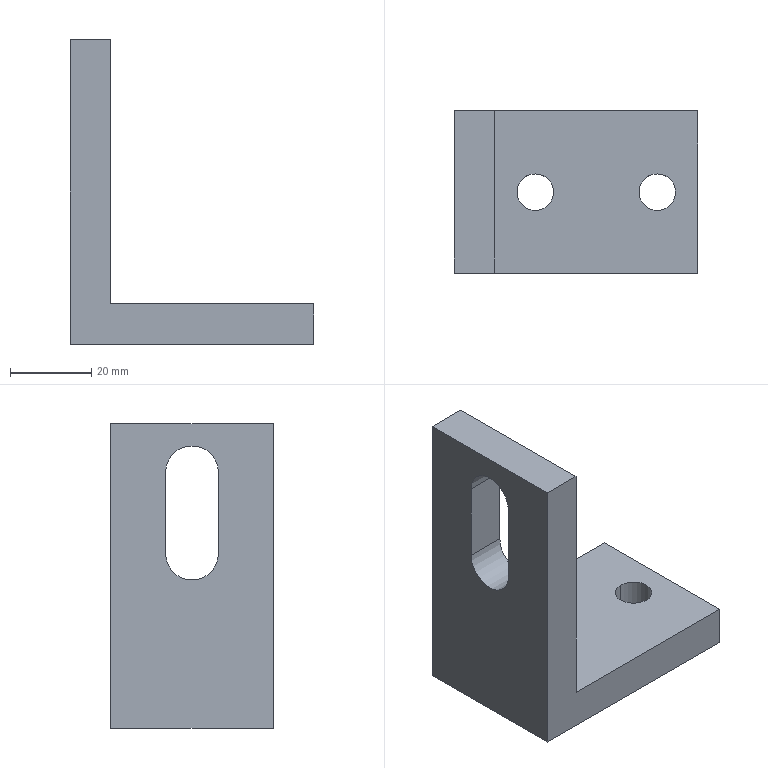Component | SolidWorks | KSD171005A-01-01-44-1 | 1 solid | 16 faces | box 60 x 40 x 75 mm | volume 44800 mm3 | plane 10 | cylinder 6 | commonest cylinder face diameters 9 x4 13 x2
build123d program:
from build123d import *

# Parameters (mm, degrees)
BOSS_EXTRUDE1_DEPTH      = 40
F_9_0_9_DIAMETER_HOLE1_D = 9
CUT_EXTRUDE1_DEPTH       = 105.043


with BuildPart() as part:
    # Sketch1 → Boss-Extrude1 (new body)
    with BuildSketch(Plane.XY):
        Polygon((0, 0), (75, 0), (75, -10), (10, -10), (10, -60), (0, -60), align=None)
    extrude(amount=BOSS_EXTRUDE1_DEPTH)

    # 9.0 _9_ Diameter Hole1 (through all)
    with Locations(Plane(origin=(10, 0, 0), x_dir=(0, 0, -1), z_dir=(1, 0, 0))):
        with Locations((-20, -20), (-20, -50)):
            Hole(F_9_0_9_DIAMETER_HOLE1_D / 2)

    # Sketch4 → Cut-Extrude1 (cut, through all)
    with BuildSketch(Plane(origin=(0, 0, 0), x_dir=(1, 0, 0), z_dir=(0, 1, 0))):
        with BuildLine():
            Line((63, -26.5), (43, -26.5))
            ThreePointArc((43, -26.5), (36.5, -20), (43, -13.5))
            Line((43, -13.5), (63, -13.5))
            ThreePointArc((63, -13.5), (69.5, -20), (63, -26.5))
        make_face()
    extrude(amount=-CUT_EXTRUDE1_DEPTH, mode=Mode.SUBTRACT)


solid = part.part

# Placed as in the assembly
solid = solid.moved(Location((32.889, -4.27, 568), (90, 0, 90)))
STEP:
#1=COLOUR_RGB('',0.7922,0.8196,0.9333);
#2=FILL_AREA_STYLE_COLOUR('',#1);
#3=FILL_AREA_STYLE('',(#2));
#4=SURFACE_STYLE_FILL_AREA(#3);
#5=SURFACE_SIDE_STYLE('',(#4));
#6=SURFACE_STYLE_USAGE(.BOTH.,#5);
#7=PRESENTATION_STYLE_ASSIGNMENT((#6));
#8=CARTESIAN_POINT('',(2.082,-1.133,22.362));
#9=VERTEX_POINT('',#8);
#10=CARTESIAN_POINT('',(2.082,-0.7784,22.362));
#11=VERTEX_POINT('',#10);
#12=CARTESIAN_POINT('',(2.082,-0.9555,22.362));
#13=DIRECTION('',(0.,0.,1.));
#14=DIRECTION('',(0.,1.,0.));
#15=AXIS2_PLACEMENT_3D('',#12,#13,#14);
#16=CIRCLE('',#15,0.1772);
#17=EDGE_CURVE('',#9,#11,#16,.T.);
#18=ORIENTED_EDGE('',*,*,#17,.F.);
#19=CARTESIAN_POINT('',(2.082,-1.133,22.756));
#20=VERTEX_POINT('',#19);
#21=CARTESIAN_POINT('',(2.082,-1.133,22.756));
#22=DIRECTION('',(0.,0.,1.));
#23=VECTOR('',#22,39.37);
#24=LINE('',#21,#23);
#25=EDGE_CURVE('',#9,#20,#24,.T.);
#26=ORIENTED_EDGE('',*,*,#25,.T.);
#27=CARTESIAN_POINT('',(2.082,-0.7784,22.756));
#28=VERTEX_POINT('',#27);
#29=CARTESIAN_POINT('',(2.082,-0.9555,22.756));
#30=DIRECTION('',(0.,0.,1.));
#31=DIRECTION('',(0.,1.,0.));
#32=AXIS2_PLACEMENT_3D('',#29,#30,#31);
#33=CIRCLE('',#32,0.1772);
#34=EDGE_CURVE('',#20,#28,#33,.T.);
#35=ORIENTED_EDGE('',*,*,#34,.T.);
#36=CARTESIAN_POINT('',(2.082,-0.7784,22.756));
#37=DIRECTION('',(0.,0.,1.));
#38=VECTOR('',#37,39.37);
#39=LINE('',#36,#38);
#40=EDGE_CURVE('',#11,#28,#39,.T.);
#41=ORIENTED_EDGE('',*,*,#40,.F.);
#42=EDGE_LOOP('',(#18,#26,#35,#41));
#43=FACE_OUTER_BOUND('',#42,.T.);
#44=CARTESIAN_POINT('',(2.082,-0.9555,22.756));
#45=DIRECTION('',(0.,0.,1.));
#46=DIRECTION('',(0.,1.,0.));
#47=AXIS2_PLACEMENT_3D('',#44,#45,#46);
#48=CYLINDRICAL_SURFACE('',#47,0.1772);
#49=ADVANCED_FACE('',(#43),#48,.F.);
#50=CARTESIAN_POINT('',(3.263,-1.133,22.362));
#51=VERTEX_POINT('',#50);
#52=CARTESIAN_POINT('',(3.263,-0.7784,22.362));
#53=VERTEX_POINT('',#52);
#54=CARTESIAN_POINT('',(3.263,-0.9555,22.362));
#55=DIRECTION('',(0.,0.,1.));
#56=DIRECTION('',(0.,1.,0.));
#57=AXIS2_PLACEMENT_3D('',#54,#55,#56);
#58=CIRCLE('',#57,0.1772);
#59=EDGE_CURVE('',#51,#53,#58,.T.);
#60=ORIENTED_EDGE('',*,*,#59,.F.);
#61=CARTESIAN_POINT('',(3.263,-1.133,22.756));
#62=VERTEX_POINT('',#61);
#63=CARTESIAN_POINT('',(3.263,-1.133,22.756));
#64=DIRECTION('',(0.,0.,1.));
#65=VECTOR('',#64,39.37);
#66=LINE('',#63,#65);
#67=EDGE_CURVE('',#51,#62,#66,.T.);
#68=ORIENTED_EDGE('',*,*,#67,.T.);
#69=CARTESIAN_POINT('',(3.263,-0.7784,22.756));
#70=VERTEX_POINT('',#69);
#71=CARTESIAN_POINT('',(3.263,-0.9555,22.756));
#72=DIRECTION('',(0.,0.,1.));
#73=DIRECTION('',(0.,1.,0.));
#74=AXIS2_PLACEMENT_3D('',#71,#72,#73);
#75=CIRCLE('',#74,0.1772);
#76=EDGE_CURVE('',#62,#70,#75,.T.);
#77=ORIENTED_EDGE('',*,*,#76,.T.);
#78=CARTESIAN_POINT('',(3.263,-0.7784,22.756));
#79=DIRECTION('',(0.,0.,1.));
#80=VECTOR('',#79,39.37);
#81=LINE('',#78,#80);
#82=EDGE_CURVE('',#53,#70,#81,.T.);
#83=ORIENTED_EDGE('',*,*,#82,.F.);
#84=EDGE_LOOP('',(#60,#68,#77,#83));
#85=FACE_OUTER_BOUND('',#84,.T.);
#86=CARTESIAN_POINT('',(3.263,-0.9555,22.756));
#87=DIRECTION('',(0.,0.,1.));
#88=DIRECTION('',(0.,1.,0.));
#89=AXIS2_PLACEMENT_3D('',#86,#87,#88);
#90=CYLINDRICAL_SURFACE('',#89,0.1772);
#91=ADVANCED_FACE('',(#85),#90,.F.);
#92=CARTESIAN_POINT('',(3.263,-0.9555,22.756));
#93=DIRECTION('',(0.,0.,1.));
#94=DIRECTION('',(0.,1.,0.));
#95=AXIS2_PLACEMENT_3D('',#92,#93,#94);
#96=CIRCLE('',#95,0.1772);
#97=EDGE_CURVE('',#70,#62,#96,.T.);
#98=ORIENTED_EDGE('',*,*,#97,.F.);
#99=ORIENTED_EDGE('',*,*,#76,.F.);
#100=EDGE_LOOP('',(#98,#99));
#101=FACE_BOUND('',#100,.T.);
#102=CARTESIAN_POINT('',(3.657,-0.1681,22.756));
#103=VERTEX_POINT('',#102);
#104=CARTESIAN_POINT('',(1.689,-0.1681,22.756));
#105=VERTEX_POINT('',#104);
#106=CARTESIAN_POINT('',(1.689,-0.1681,22.756));
#107=DIRECTION('',(-1.,0.,0.));
#108=VECTOR('',#107,39.37);
#109=LINE('',#106,#108);
#110=EDGE_CURVE('',#103,#105,#109,.T.);
#111=ORIENTED_EDGE('',*,*,#110,.T.);
#112=CARTESIAN_POINT('',(1.689,-1.743,22.756));
#113=VERTEX_POINT('',#112);
#114=CARTESIAN_POINT('',(1.689,-1.743,22.756));
#115=DIRECTION('',(0.,1.,-0.));
#116=VECTOR('',#115,39.37);
#117=LINE('',#114,#116);
#118=EDGE_CURVE('',#113,#105,#117,.T.);
#119=ORIENTED_EDGE('',*,*,#118,.F.);
#120=CARTESIAN_POINT('',(3.657,-1.743,22.756));
#121=VERTEX_POINT('',#120);
#122=CARTESIAN_POINT('',(1.689,-1.743,22.756));
#123=DIRECTION('',(-1.,0.,0.));
#124=VECTOR('',#123,39.37);
#125=LINE('',#122,#124);
#126=EDGE_CURVE('',#121,#113,#125,.T.);
#127=ORIENTED_EDGE('',*,*,#126,.F.);
#128=CARTESIAN_POINT('',(3.657,-1.743,22.756));
#129=DIRECTION('',(0.,1.,-0.));
#130=VECTOR('',#129,39.37);
#131=LINE('',#128,#130);
#132=EDGE_CURVE('',#121,#103,#131,.T.);
#133=ORIENTED_EDGE('',*,*,#132,.T.);
#134=EDGE_LOOP('',(#111,#119,#127,#133));
#135=FACE_OUTER_BOUND('',#134,.T.);
#136=CARTESIAN_POINT('',(2.082,-0.9555,22.756));
#137=DIRECTION('',(0.,0.,1.));
#138=DIRECTION('',(0.,1.,0.));
#139=AXIS2_PLACEMENT_3D('',#136,#137,#138);
#140=CIRCLE('',#139,0.1772);
#141=EDGE_CURVE('',#28,#20,#140,.T.);
#142=ORIENTED_EDGE('',*,*,#141,.F.);
#143=ORIENTED_EDGE('',*,*,#34,.F.);
#144=EDGE_LOOP('',(#142,#143));
#145=FACE_BOUND('',#144,.T.);
#146=CARTESIAN_POINT('',(1.689,-1.743,22.756));
#147=DIRECTION('',(-0.,-0.,-1.));
#148=DIRECTION('',(1.,-0.,-0.));
#149=AXIS2_PLACEMENT_3D('',#146,#147,#148);
#150=PLANE('',#149);
#151=ADVANCED_FACE('',(#101,#135,#145),#150,.F.);
#152=CARTESIAN_POINT('',(2.082,-0.9555,22.362));
#153=DIRECTION('',(0.,0.,1.));
#154=DIRECTION('',(0.,1.,0.));
#155=AXIS2_PLACEMENT_3D('',#152,#153,#154);
#156=CIRCLE('',#155,0.1772);
#157=EDGE_CURVE('',#11,#9,#156,.T.);
#158=ORIENTED_EDGE('',*,*,#157,.T.);
#159=ORIENTED_EDGE('',*,*,#17,.T.);
#160=EDGE_LOOP('',(#158,#159));
#161=FACE_BOUND('',#160,.T.);
#162=CARTESIAN_POINT('',(3.263,-0.9555,22.362));
#163=DIRECTION('',(0.,0.,1.));
#164=DIRECTION('',(0.,1.,0.));
#165=AXIS2_PLACEMENT_3D('',#162,#163,#164);
#166=CIRCLE('',#165,0.1772);
#167=EDGE_CURVE('',#53,#51,#166,.T.);
#168=ORIENTED_EDGE('',*,*,#167,.T.);
#169=ORIENTED_EDGE('',*,*,#59,.T.);
#170=EDGE_LOOP('',(#168,#169));
#171=FACE_BOUND('',#170,.T.);
#172=CARTESIAN_POINT('',(1.295,-0.1681,22.362));
#173=VERTEX_POINT('',#172);
#174=CARTESIAN_POINT('',(3.657,-0.1681,22.362));
#175=VERTEX_POINT('',#174);
#176=CARTESIAN_POINT('',(1.295,-0.1681,22.362));
#177=DIRECTION('',(1.,-0.,0.));
#178=VECTOR('',#177,39.37);
#179=LINE('',#176,#178);
#180=EDGE_CURVE('',#173,#175,#179,.T.);
#181=ORIENTED_EDGE('',*,*,#180,.T.);
#182=CARTESIAN_POINT('',(3.657,-1.743,22.362));
#183=VERTEX_POINT('',#182);
#184=CARTESIAN_POINT('',(3.657,-1.743,22.362));
#185=DIRECTION('',(0.,1.,-0.));
#186=VECTOR('',#185,39.37);
#187=LINE('',#184,#186);
#188=EDGE_CURVE('',#183,#175,#187,.T.);
#189=ORIENTED_EDGE('',*,*,#188,.F.);
#190=CARTESIAN_POINT('',(1.295,-1.743,22.362));
#191=VERTEX_POINT('',#190);
#192=CARTESIAN_POINT('',(1.295,-1.743,22.362));
#193=DIRECTION('',(1.,-0.,0.));
#194=VECTOR('',#193,39.37);
#195=LINE('',#192,#194);
#196=EDGE_CURVE('',#191,#183,#195,.T.);
#197=ORIENTED_EDGE('',*,*,#196,.F.);
#198=CARTESIAN_POINT('',(1.295,-1.743,22.362));
#199=DIRECTION('',(0.,1.,-0.));
#200=VECTOR('',#199,39.37);
#201=LINE('',#198,#200);
#202=EDGE_CURVE('',#191,#173,#201,.T.);
#203=ORIENTED_EDGE('',*,*,#202,.T.);
#204=EDGE_LOOP('',(#181,#189,#197,#203));
#205=FACE_OUTER_BOUND('',#204,.T.);
#206=CARTESIAN_POINT('',(1.295,-1.743,22.362));
#207=DIRECTION('',(-0.,0.,1.));
#208=DIRECTION('',(-1.,0.,-0.));
#209=AXIS2_PLACEMENT_3D('',#206,#207,#208);
#210=PLANE('',#209);
#211=ADVANCED_FACE('',(#161,#171,#205),#210,.F.);
#212=CARTESIAN_POINT('',(3.657,-0.1681,22.756));
#213=DIRECTION('',(0.,0.,1.));
#214=VECTOR('',#213,39.37);
#215=LINE('',#212,#214);
#216=EDGE_CURVE('',#175,#103,#215,.T.);
#217=ORIENTED_EDGE('',*,*,#216,.T.);
#218=ORIENTED_EDGE('',*,*,#132,.F.);
#219=CARTESIAN_POINT('',(3.657,-1.743,22.756));
#220=DIRECTION('',(0.,0.,1.));
#221=VECTOR('',#220,39.37);
#222=LINE('',#219,#221);
#223=EDGE_CURVE('',#183,#121,#222,.T.);
#224=ORIENTED_EDGE('',*,*,#223,.F.);
#225=ORIENTED_EDGE('',*,*,#188,.T.);
#226=EDGE_LOOP('',(#217,#218,#224,#225));
#227=FACE_OUTER_BOUND('',#226,.T.);
#228=CARTESIAN_POINT('',(3.657,-1.743,22.756));
#229=DIRECTION('',(-1.,0.,0.));
#230=DIRECTION('',(-0.,-1.,0.));
#231=AXIS2_PLACEMENT_3D('',#228,#229,#230);
#232=PLANE('',#231);
#233=ADVANCED_FACE('',(#227),#232,.F.);
#234=CARTESIAN_POINT('',(1.689,-1.211,24.055));
#235=VERTEX_POINT('',#234);
#236=CARTESIAN_POINT('',(1.689,-1.211,24.843));
#237=VERTEX_POINT('',#236);
#238=CARTESIAN_POINT('',(1.689,-1.211,25.315));
#239=DIRECTION('',(0.,0.,1.));
#240=VECTOR('',#239,39.37);
#241=LINE('',#238,#240);
#242=EDGE_CURVE('',#235,#237,#241,.T.);
#243=ORIENTED_EDGE('',*,*,#242,.T.);
#244=CARTESIAN_POINT('',(1.689,-0.6996,24.843));
#245=VERTEX_POINT('',#244);
#246=CARTESIAN_POINT('',(1.689,-0.9555,24.843));
#247=DIRECTION('',(-1.,0.,0.));
#248=DIRECTION('',(0.,0.,-1.));
#249=AXIS2_PLACEMENT_3D('',#246,#247,#248);
#250=CIRCLE('',#249,0.2559);
#251=EDGE_CURVE('',#237,#245,#250,.T.);
#252=ORIENTED_EDGE('',*,*,#251,.T.);
#253=CARTESIAN_POINT('',(1.689,-0.6996,24.055));
#254=VERTEX_POINT('',#253);
#255=CARTESIAN_POINT('',(1.689,-0.6996,25.315));
#256=DIRECTION('',(-0.,-0.,-1.));
#257=VECTOR('',#256,39.37);
#258=LINE('',#255,#257);
#259=EDGE_CURVE('',#245,#254,#258,.T.);
#260=ORIENTED_EDGE('',*,*,#259,.T.);
#261=CARTESIAN_POINT('',(1.689,-0.9555,24.055));
#262=DIRECTION('',(-1.,0.,0.));
#263=DIRECTION('',(0.,0.,-1.));
#264=AXIS2_PLACEMENT_3D('',#261,#262,#263);
#265=CIRCLE('',#264,0.2559);
#266=EDGE_CURVE('',#254,#235,#265,.T.);
#267=ORIENTED_EDGE('',*,*,#266,.T.);
#268=EDGE_LOOP('',(#243,#252,#260,#267));
#269=FACE_BOUND('',#268,.T.);
#270=CARTESIAN_POINT('',(1.689,-0.1681,25.315));
#271=VERTEX_POINT('',#270);
#272=CARTESIAN_POINT('',(1.689,-0.1681,25.315));
#273=DIRECTION('',(0.,0.,1.));
#274=VECTOR('',#273,39.37);
#275=LINE('',#272,#274);
#276=EDGE_CURVE('',#105,#271,#275,.T.);
#277=ORIENTED_EDGE('',*,*,#276,.T.);
#278=CARTESIAN_POINT('',(1.689,-1.743,25.315));
#279=VERTEX_POINT('',#278);
#280=CARTESIAN_POINT('',(1.689,-1.743,25.315));
#281=DIRECTION('',(0.,1.,-0.));
#282=VECTOR('',#281,39.37);
#283=LINE('',#280,#282);
#284=EDGE_CURVE('',#279,#271,#283,.T.);
#285=ORIENTED_EDGE('',*,*,#284,.F.);
#286=CARTESIAN_POINT('',(1.689,-1.743,25.315));
#287=DIRECTION('',(0.,0.,1.));
#288=VECTOR('',#287,39.37);
#289=LINE('',#286,#288);
#290=EDGE_CURVE('',#113,#279,#289,.T.);
#291=ORIENTED_EDGE('',*,*,#290,.F.);
#292=ORIENTED_EDGE('',*,*,#118,.T.);
#293=EDGE_LOOP('',(#277,#285,#291,#292));
#294=FACE_OUTER_BOUND('',#293,.T.);
#295=CARTESIAN_POINT('',(1.689,-1.743,25.315));
#296=DIRECTION('',(-1.,0.,0.));
#297=DIRECTION('',(-0.,-0.,-1.));
#298=AXIS2_PLACEMENT_3D('',#295,#296,#297);
#299=PLANE('',#298);
#300=ADVANCED_FACE('',(#269,#294),#299,.F.);
#301=CARTESIAN_POINT('',(1.295,-0.1681,25.315));
#302=VERTEX_POINT('',#301);
#303=CARTESIAN_POINT('',(1.295,-0.1681,25.315));
#304=DIRECTION('',(-1.,0.,0.));
#305=VECTOR('',#304,39.37);
#306=LINE('',#303,#305);
#307=EDGE_CURVE('',#271,#302,#306,.T.);
#308=ORIENTED_EDGE('',*,*,#307,.T.);
#309=CARTESIAN_POINT('',(1.295,-1.743,25.315));
#310=VERTEX_POINT('',#309);
#311=CARTESIAN_POINT('',(1.295,-1.743,25.315));
#312=DIRECTION('',(0.,1.,-0.));
#313=VECTOR('',#312,39.37);
#314=LINE('',#311,#313);
#315=EDGE_CURVE('',#310,#302,#314,.T.);
#316=ORIENTED_EDGE('',*,*,#315,.F.);
#317=CARTESIAN_POINT('',(1.295,-1.743,25.315));
#318=DIRECTION('',(-1.,0.,0.));
#319=VECTOR('',#318,39.37);
#320=LINE('',#317,#319);
#321=EDGE_CURVE('',#279,#310,#320,.T.);
#322=ORIENTED_EDGE('',*,*,#321,.F.);
#323=ORIENTED_EDGE('',*,*,#284,.T.);
#324=EDGE_LOOP('',(#308,#316,#322,#323));
#325=FACE_OUTER_BOUND('',#324,.T.);
#326=CARTESIAN_POINT('',(1.295,-1.743,25.315));
#327=DIRECTION('',(-0.,-0.,-1.));
#328=DIRECTION('',(-0.,-1.,0.));
#329=AXIS2_PLACEMENT_3D('',#326,#327,#328);
#330=PLANE('',#329);
#331=ADVANCED_FACE('',(#325),#330,.F.);
#332=CARTESIAN_POINT('',(1.295,-0.6996,24.843));
#333=VERTEX_POINT('',#332);
#334=CARTESIAN_POINT('',(1.295,-0.6996,24.055));
#335=VERTEX_POINT('',#334);
#336=CARTESIAN_POINT('',(1.295,-0.6996,24.843));
#337=DIRECTION('',(-0.,-0.,-1.));
#338=VECTOR('',#337,39.37);
#339=LINE('',#336,#338);
#340=EDGE_CURVE('',#333,#335,#339,.T.);
#341=ORIENTED_EDGE('',*,*,#340,.F.);
#342=CARTESIAN_POINT('',(1.295,-1.211,24.843));
#343=VERTEX_POINT('',#342);
#344=CARTESIAN_POINT('',(1.295,-0.9555,24.843));
#345=DIRECTION('',(-1.,0.,0.));
#346=DIRECTION('',(0.,-1.,0.));
#347=AXIS2_PLACEMENT_3D('',#344,#345,#346);
#348=CIRCLE('',#347,0.2559);
#349=EDGE_CURVE('',#343,#333,#348,.T.);
#350=ORIENTED_EDGE('',*,*,#349,.F.);
#351=CARTESIAN_POINT('',(1.295,-1.211,24.055));
#352=VERTEX_POINT('',#351);
#353=CARTESIAN_POINT('',(1.295,-1.211,24.843));
#354=DIRECTION('',(0.,0.,1.));
#355=VECTOR('',#354,39.37);
#356=LINE('',#353,#355);
#357=EDGE_CURVE('',#352,#343,#356,.T.);
#358=ORIENTED_EDGE('',*,*,#357,.F.);
#359=CARTESIAN_POINT('',(1.295,-0.9555,24.055));
#360=DIRECTION('',(-1.,0.,0.));
#361=DIRECTION('',(0.,-1.,0.));
#362=AXIS2_PLACEMENT_3D('',#359,#360,#361);
#363=CIRCLE('',#362,0.2559);
#364=EDGE_CURVE('',#335,#352,#363,.T.);
#365=ORIENTED_EDGE('',*,*,#364,.F.);
#366=EDGE_LOOP('',(#341,#350,#358,#365));
#367=FACE_BOUND('',#366,.T.);
#368=CARTESIAN_POINT('',(1.295,-0.1681,22.362));
#369=DIRECTION('',(-0.,-0.,-1.));
#370=VECTOR('',#369,39.37);
#371=LINE('',#368,#370);
#372=EDGE_CURVE('',#302,#173,#371,.T.);
#373=ORIENTED_EDGE('',*,*,#372,.T.);
#374=ORIENTED_EDGE('',*,*,#202,.F.);
#375=CARTESIAN_POINT('',(1.295,-1.743,22.362));
#376=DIRECTION('',(-0.,-0.,-1.));
#377=VECTOR('',#376,39.37);
#378=LINE('',#375,#377);
#379=EDGE_CURVE('',#310,#191,#378,.T.);
#380=ORIENTED_EDGE('',*,*,#379,.F.);
#381=ORIENTED_EDGE('',*,*,#315,.T.);
#382=EDGE_LOOP('',(#373,#374,#380,#381));
#383=FACE_OUTER_BOUND('',#382,.T.);
#384=CARTESIAN_POINT('',(1.295,-1.743,22.362));
#385=DIRECTION('',(1.,-0.,-0.));
#386=DIRECTION('',(0.,1.,-0.));
#387=AXIS2_PLACEMENT_3D('',#384,#385,#386);
#388=PLANE('',#387);
#389=ADVANCED_FACE('',(#367,#383),#388,.F.);
#390=ORIENTED_EDGE('',*,*,#196,.T.);
#391=ORIENTED_EDGE('',*,*,#223,.T.);
#392=ORIENTED_EDGE('',*,*,#126,.T.);
#393=ORIENTED_EDGE('',*,*,#290,.T.);
#394=ORIENTED_EDGE('',*,*,#321,.T.);
#395=ORIENTED_EDGE('',*,*,#379,.T.);
#396=EDGE_LOOP('',(#390,#391,#392,#393,#394,#395));
#397=FACE_OUTER_BOUND('',#396,.T.);
#398=CARTESIAN_POINT('',(1.295,-1.743,22.362));
#399=DIRECTION('',(0.,1.,-0.));
#400=DIRECTION('',(-0.,-0.,-1.));
#401=AXIS2_PLACEMENT_3D('',#398,#399,#400);
#402=PLANE('',#401);
#403=ADVANCED_FACE('',(#397),#402,.F.);
#404=ORIENTED_EDGE('',*,*,#180,.F.);
#405=ORIENTED_EDGE('',*,*,#372,.F.);
#406=ORIENTED_EDGE('',*,*,#307,.F.);
#407=ORIENTED_EDGE('',*,*,#276,.F.);
#408=ORIENTED_EDGE('',*,*,#110,.F.);
#409=ORIENTED_EDGE('',*,*,#216,.F.);
#410=EDGE_LOOP('',(#404,#405,#406,#407,#408,#409));
#411=FACE_OUTER_BOUND('',#410,.T.);
#412=CARTESIAN_POINT('',(1.295,-0.1681,22.362));
#413=DIRECTION('',(0.,1.,-0.));
#414=DIRECTION('',(-0.,-0.,-1.));
#415=AXIS2_PLACEMENT_3D('',#412,#413,#414);
#416=PLANE('',#415);
#417=ADVANCED_FACE('',(#411),#416,.T.);
#418=ORIENTED_EDGE('',*,*,#67,.F.);
#419=ORIENTED_EDGE('',*,*,#167,.F.);
#420=ORIENTED_EDGE('',*,*,#82,.T.);
#421=ORIENTED_EDGE('',*,*,#97,.T.);
#422=EDGE_LOOP('',(#418,#419,#420,#421));
#423=FACE_OUTER_BOUND('',#422,.T.);
#424=CARTESIAN_POINT('',(3.263,-0.9555,22.756));
#425=DIRECTION('',(0.,0.,1.));
#426=DIRECTION('',(0.,1.,0.));
#427=AXIS2_PLACEMENT_3D('',#424,#425,#426);
#428=CYLINDRICAL_SURFACE('',#427,0.1772);
#429=ADVANCED_FACE('',(#423),#428,.F.);
#430=ORIENTED_EDGE('',*,*,#25,.F.);
#431=ORIENTED_EDGE('',*,*,#157,.F.);
#432=ORIENTED_EDGE('',*,*,#40,.T.);
#433=ORIENTED_EDGE('',*,*,#141,.T.);
#434=EDGE_LOOP('',(#430,#431,#432,#433));
#435=FACE_OUTER_BOUND('',#434,.T.);
#436=CARTESIAN_POINT('',(2.082,-0.9555,22.756));
#437=DIRECTION('',(0.,0.,1.));
#438=DIRECTION('',(0.,1.,0.));
#439=AXIS2_PLACEMENT_3D('',#436,#437,#438);
#440=CYLINDRICAL_SURFACE('',#439,0.1772);
#441=ADVANCED_FACE('',(#435),#440,.F.);
#442=CARTESIAN_POINT('',(3.657,-1.211,24.843));
#443=DIRECTION('',(-1.,0.,0.));
#444=VECTOR('',#443,39.37);
#445=LINE('',#442,#444);
#446=EDGE_CURVE('',#237,#343,#445,.T.);
#447=ORIENTED_EDGE('',*,*,#446,.T.);
#448=ORIENTED_EDGE('',*,*,#349,.T.);
#449=CARTESIAN_POINT('',(3.657,-0.6996,24.843));
#450=DIRECTION('',(-1.,0.,0.));
#451=VECTOR('',#450,39.37);
#452=LINE('',#449,#451);
#453=EDGE_CURVE('',#245,#333,#452,.T.);
#454=ORIENTED_EDGE('',*,*,#453,.F.);
#455=ORIENTED_EDGE('',*,*,#251,.F.);
#456=EDGE_LOOP('',(#447,#448,#454,#455));
#457=FACE_OUTER_BOUND('',#456,.T.);
#458=CARTESIAN_POINT('',(3.657,-0.9555,24.843));
#459=DIRECTION('',(-1.,0.,0.));
#460=DIRECTION('',(0.,-1.,0.));
#461=AXIS2_PLACEMENT_3D('',#458,#459,#460);
#462=CYLINDRICAL_SURFACE('',#461,0.2559);
#463=ADVANCED_FACE('',(#457),#462,.F.);
#464=CARTESIAN_POINT('',(3.657,-1.211,24.055));
#465=DIRECTION('',(-1.,0.,0.));
#466=VECTOR('',#465,39.37);
#467=LINE('',#464,#466);
#468=EDGE_CURVE('',#235,#352,#467,.T.);
#469=ORIENTED_EDGE('',*,*,#468,.T.);
#470=ORIENTED_EDGE('',*,*,#357,.T.);
#471=ORIENTED_EDGE('',*,*,#446,.F.);
#472=ORIENTED_EDGE('',*,*,#242,.F.);
#473=EDGE_LOOP('',(#469,#470,#471,#472));
#474=FACE_OUTER_BOUND('',#473,.T.);
#475=CARTESIAN_POINT('',(3.657,-1.211,24.843));
#476=DIRECTION('',(-0.,-1.,0.));
#477=DIRECTION('',(0.,0.,1.));
#478=AXIS2_PLACEMENT_3D('',#475,#476,#477);
#479=PLANE('',#478);
#480=ADVANCED_FACE('',(#474),#479,.F.);
#481=CARTESIAN_POINT('',(3.657,-0.6996,24.055));
#482=DIRECTION('',(-1.,0.,0.));
#483=VECTOR('',#482,39.37);
#484=LINE('',#481,#483);
#485=EDGE_CURVE('',#254,#335,#484,.T.);
#486=ORIENTED_EDGE('',*,*,#485,.T.);
#487=ORIENTED_EDGE('',*,*,#364,.T.);
#488=ORIENTED_EDGE('',*,*,#468,.F.);
#489=ORIENTED_EDGE('',*,*,#266,.F.);
#490=EDGE_LOOP('',(#486,#487,#488,#489));
#491=FACE_OUTER_BOUND('',#490,.T.);
#492=CARTESIAN_POINT('',(3.657,-0.9555,24.055));
#493=DIRECTION('',(-1.,0.,0.));
#494=DIRECTION('',(0.,-1.,0.));
#495=AXIS2_PLACEMENT_3D('',#492,#493,#494);
#496=CYLINDRICAL_SURFACE('',#495,0.2559);
#497=ADVANCED_FACE('',(#491),#496,.F.);
#498=ORIENTED_EDGE('',*,*,#453,.T.);
#499=ORIENTED_EDGE('',*,*,#340,.T.);
#500=ORIENTED_EDGE('',*,*,#485,.F.);
#501=ORIENTED_EDGE('',*,*,#259,.F.);
#502=EDGE_LOOP('',(#498,#499,#500,#501));
#503=FACE_OUTER_BOUND('',#502,.T.);
#504=CARTESIAN_POINT('',(3.657,-0.6996,24.843));
#505=DIRECTION('',(0.,1.,-0.));
#506=DIRECTION('',(-0.,-0.,-1.));
#507=AXIS2_PLACEMENT_3D('',#504,#505,#506);
#508=PLANE('',#507);
#509=ADVANCED_FACE('',(#503),#508,.F.);
#510=CLOSED_SHELL('',(#49,#91,#151,#211,#233,#300,#331,#389,#403,#417,#429,#441,#463,#480,#497,#509));
#511=MANIFOLD_SOLID_BREP('',#510);
#512=STYLED_ITEM('',(#7),#511);
#513=PRESENTATION_LAYER_ASSIGNMENT('','',(#512));
#514=(LENGTH_UNIT()NAMED_UNIT(*)SI_UNIT($,.METRE.));
#515=LENGTH_MEASURE_WITH_UNIT(LENGTH_MEASURE(0.0254),#514);
#516=DIMENSIONAL_EXPONENTS(1.,0.,0.,0.,0.,0.,0.);
#517=(CONVERSION_BASED_UNIT('',#515)LENGTH_UNIT()NAMED_UNIT(#516));
#518=UNCERTAINTY_MEASURE_WITH_UNIT(LENGTH_MEASURE(0.00001),#517,'','');
#519=(NAMED_UNIT(*)PLANE_ANGLE_UNIT()SI_UNIT($,.RADIAN.));
#520=(NAMED_UNIT(*)SI_UNIT($,.STERADIAN.)SOLID_ANGLE_UNIT());
#521=(GEOMETRIC_REPRESENTATION_CONTEXT(3)GLOBAL_UNCERTAINTY_ASSIGNED_CONTEXT((#518))GLOBAL_UNIT_ASSIGNED_CONTEXT((#517,#519,#520))REPRESENTATION_CONTEXT('',''));
#522=MECHANICAL_DESIGN_GEOMETRIC_PRESENTATION_REPRESENTATION('',(#512),#521);
#523=CARTESIAN_POINT('',(0.,0.,0.));
#524=DIRECTION('',(0.,0.,1.));
#525=DIRECTION('',(1.,0.,0.));
#526=AXIS2_PLACEMENT_3D('',#523,#524,#525);
#527=(LENGTH_UNIT()NAMED_UNIT(*)SI_UNIT($,.METRE.));
#528=LENGTH_MEASURE_WITH_UNIT(LENGTH_MEASURE(0.0254),#527);
#529=DIMENSIONAL_EXPONENTS(1.,0.,0.,0.,0.,0.,0.);
#530=(CONVERSION_BASED_UNIT('',#528)LENGTH_UNIT()NAMED_UNIT(#529));
#531=UNCERTAINTY_MEASURE_WITH_UNIT(LENGTH_MEASURE(0.00001),#530,'','');
#532=(NAMED_UNIT(*)PLANE_ANGLE_UNIT()SI_UNIT($,.RADIAN.));
#533=(NAMED_UNIT(*)SI_UNIT($,.STERADIAN.)SOLID_ANGLE_UNIT());
#534=(GEOMETRIC_REPRESENTATION_CONTEXT(3)GLOBAL_UNCERTAINTY_ASSIGNED_CONTEXT((#531))GLOBAL_UNIT_ASSIGNED_CONTEXT((#530,#532,#533))REPRESENTATION_CONTEXT('',''));
#535=ADVANCED_BREP_SHAPE_REPRESENTATION('',(#511,#526),#534);